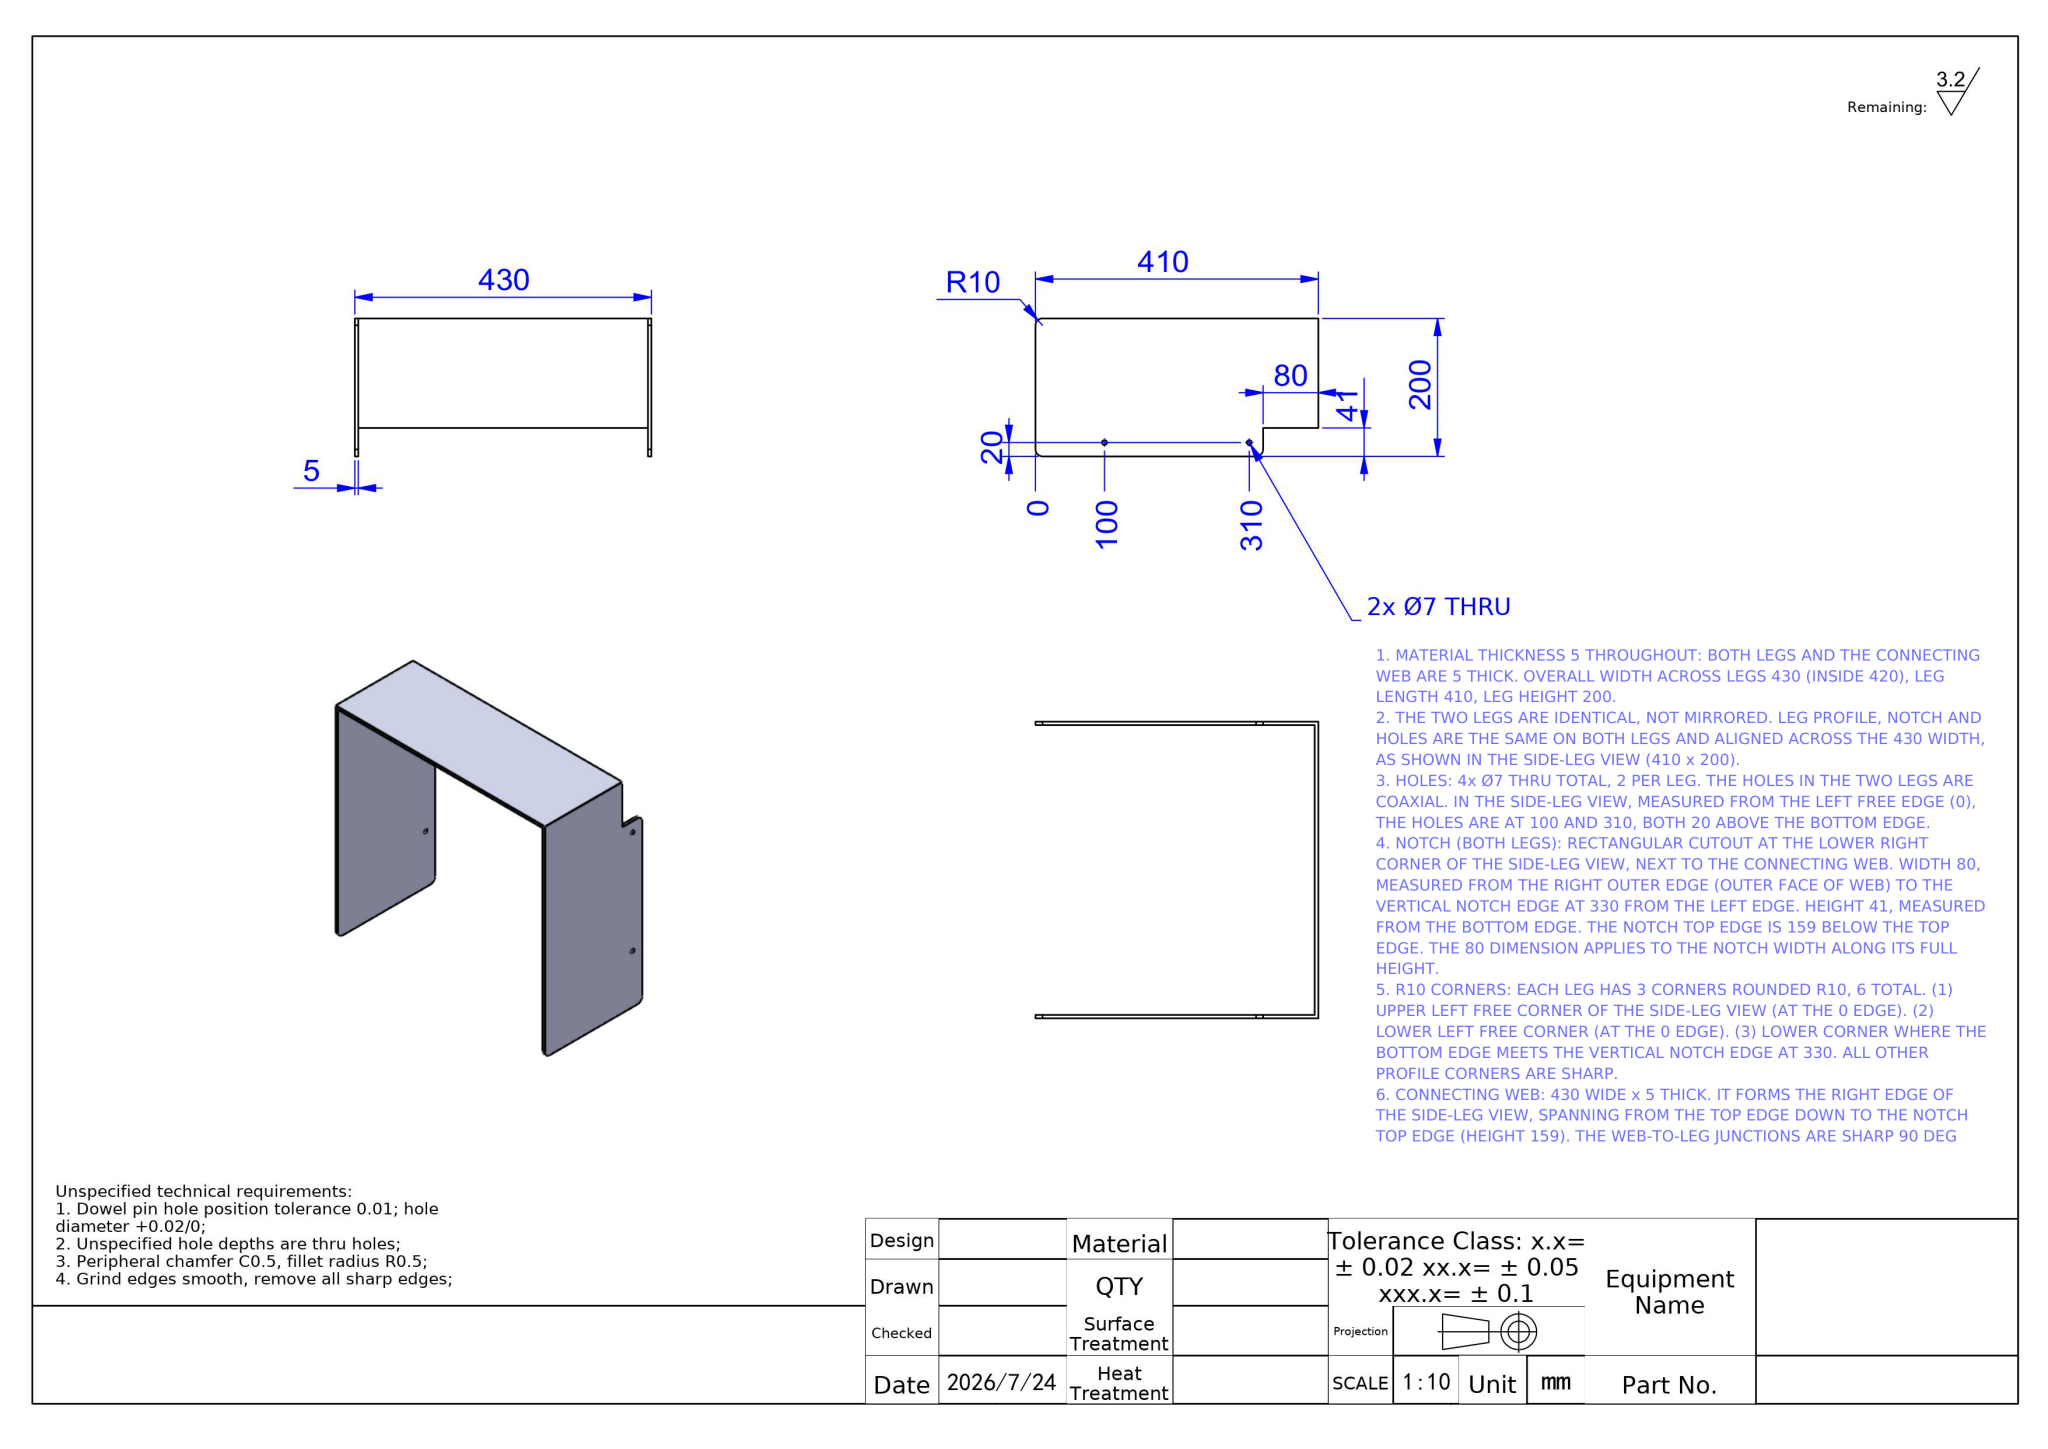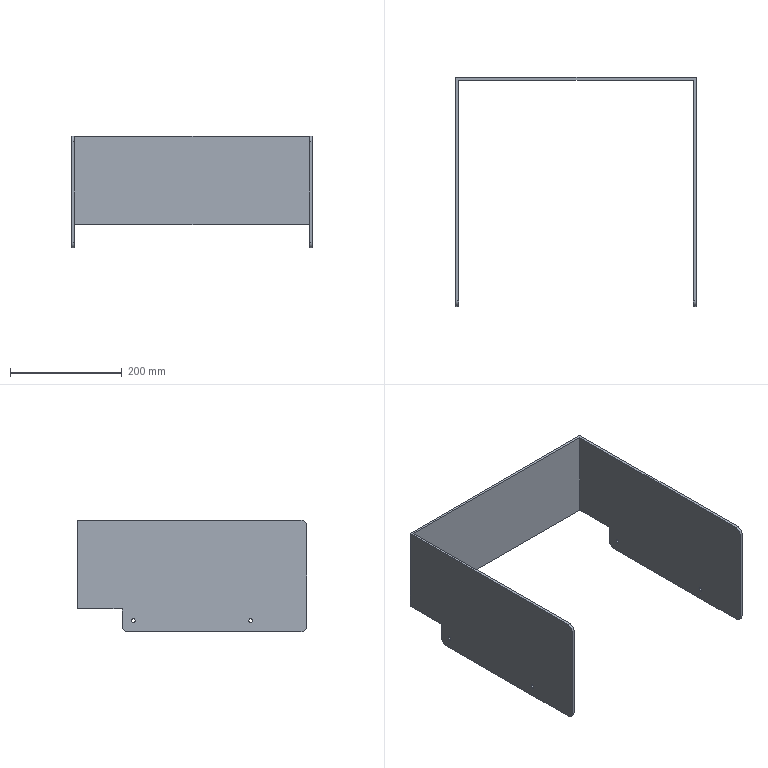Part | NX | mm | Stepped Dual-Tab U-Channel Bracket | 1 solid | 28 faces | box 430 x 410 x 200 mm | volume 1119687 mm3 | cylinder 14 | plane 14 | commonest cylinder face diameters 7 x8 20 x6
STEP:
#1=COLOUR_RGB('',0.7922,0.8196,0.9333);
#2=FILL_AREA_STYLE_COLOUR('',#1);
#3=FILL_AREA_STYLE('',(#2));
#4=SURFACE_STYLE_FILL_AREA(#3);
#5=SURFACE_SIDE_STYLE('',(#4));
#6=SURFACE_STYLE_USAGE(.BOTH.,#5);
#7=PRESENTATION_STYLE_ASSIGNMENT((#6));
#8=CARTESIAN_POINT('',(-210.,105.,-76.5));
#9=VERTEX_POINT('',#8);
#10=CARTESIAN_POINT('',(-210.,105.,-83.5));
#11=VERTEX_POINT('',#10);
#12=CARTESIAN_POINT('',(-210.,105.,-80.));
#13=DIRECTION('',(1.,0.,0.));
#14=DIRECTION('',(0.,1.,0.));
#15=AXIS2_PLACEMENT_3D('',#12,#13,#14);
#16=CIRCLE('',#15,3.5);
#17=EDGE_CURVE('',#9,#11,#16,.T.);
#18=ORIENTED_EDGE('',*,*,#17,.T.);
#19=CARTESIAN_POINT('',(-215.,105.,-83.5));
#20=VERTEX_POINT('',#19);
#21=CARTESIAN_POINT('',(-215.,105.,-83.5));
#22=DIRECTION('',(-1.,0.,0.));
#23=VECTOR('',#22,1000.);
#24=LINE('',#21,#23);
#25=EDGE_CURVE('',#11,#20,#24,.T.);
#26=ORIENTED_EDGE('',*,*,#25,.T.);
#27=CARTESIAN_POINT('',(-215.,105.,-76.5));
#28=VERTEX_POINT('',#27);
#29=CARTESIAN_POINT('',(-215.,105.,-80.));
#30=DIRECTION('',(-1.,0.,0.));
#31=DIRECTION('',(0.,0.,1.));
#32=AXIS2_PLACEMENT_3D('',#29,#30,#31);
#33=CIRCLE('',#32,3.5);
#34=EDGE_CURVE('',#20,#28,#33,.T.);
#35=ORIENTED_EDGE('',*,*,#34,.T.);
#36=CARTESIAN_POINT('',(-215.,105.,-76.5));
#37=DIRECTION('',(-1.,0.,0.));
#38=VECTOR('',#37,1000.);
#39=LINE('',#36,#38);
#40=EDGE_CURVE('',#9,#28,#39,.T.);
#41=ORIENTED_EDGE('',*,*,#40,.F.);
#42=EDGE_LOOP('',(#18,#26,#35,#41));
#43=FACE_OUTER_BOUND('',#42,.T.);
#44=CARTESIAN_POINT('',(-215.,105.,-80.));
#45=DIRECTION('',(-1.,0.,0.));
#46=DIRECTION('',(0.,0.,1.));
#47=AXIS2_PLACEMENT_3D('',#44,#45,#46);
#48=CYLINDRICAL_SURFACE('',#47,3.5);
#49=ADVANCED_FACE('',(#43),#48,.F.);
#50=CARTESIAN_POINT('',(215.,105.,-83.5));
#51=VERTEX_POINT('',#50);
#52=CARTESIAN_POINT('',(215.,105.,-76.5));
#53=VERTEX_POINT('',#52);
#54=CARTESIAN_POINT('',(215.,105.,-80.));
#55=DIRECTION('',(-1.,0.,0.));
#56=DIRECTION('',(0.,0.,1.));
#57=AXIS2_PLACEMENT_3D('',#54,#55,#56);
#58=CIRCLE('',#57,3.5);
#59=EDGE_CURVE('',#51,#53,#58,.T.);
#60=ORIENTED_EDGE('',*,*,#59,.F.);
#61=CARTESIAN_POINT('',(210.,105.,-83.5));
#62=VERTEX_POINT('',#61);
#63=CARTESIAN_POINT('',(-215.,105.,-83.5));
#64=DIRECTION('',(-1.,0.,0.));
#65=VECTOR('',#64,1000.);
#66=LINE('',#63,#65);
#67=EDGE_CURVE('',#51,#62,#66,.T.);
#68=ORIENTED_EDGE('',*,*,#67,.T.);
#69=CARTESIAN_POINT('',(210.,105.,-76.5));
#70=VERTEX_POINT('',#69);
#71=CARTESIAN_POINT('',(210.,105.,-80.));
#72=DIRECTION('',(-1.,-0.,0.));
#73=DIRECTION('',(0.,-1.,0.));
#74=AXIS2_PLACEMENT_3D('',#71,#72,#73);
#75=CIRCLE('',#74,3.5);
#76=EDGE_CURVE('',#62,#70,#75,.T.);
#77=ORIENTED_EDGE('',*,*,#76,.T.);
#78=CARTESIAN_POINT('',(-215.,105.,-76.5));
#79=DIRECTION('',(-1.,0.,0.));
#80=VECTOR('',#79,1000.);
#81=LINE('',#78,#80);
#82=EDGE_CURVE('',#53,#70,#81,.T.);
#83=ORIENTED_EDGE('',*,*,#82,.F.);
#84=EDGE_LOOP('',(#60,#68,#77,#83));
#85=FACE_OUTER_BOUND('',#84,.T.);
#86=CARTESIAN_POINT('',(-215.,105.,-80.));
#87=DIRECTION('',(-1.,0.,0.));
#88=DIRECTION('',(0.,0.,1.));
#89=AXIS2_PLACEMENT_3D('',#86,#87,#88);
#90=CYLINDRICAL_SURFACE('',#89,3.5);
#91=ADVANCED_FACE('',(#85),#90,.F.);
#92=CARTESIAN_POINT('',(215.,-105.,-83.5));
#93=VERTEX_POINT('',#92);
#94=CARTESIAN_POINT('',(215.,-105.,-76.5));
#95=VERTEX_POINT('',#94);
#96=CARTESIAN_POINT('',(215.,-105.,-80.));
#97=DIRECTION('',(-1.,0.,0.));
#98=DIRECTION('',(0.,0.,1.));
#99=AXIS2_PLACEMENT_3D('',#96,#97,#98);
#100=CIRCLE('',#99,3.5);
#101=EDGE_CURVE('',#93,#95,#100,.T.);
#102=ORIENTED_EDGE('',*,*,#101,.F.);
#103=CARTESIAN_POINT('',(210.,-105.,-83.5));
#104=VERTEX_POINT('',#103);
#105=CARTESIAN_POINT('',(-215.,-105.,-83.5));
#106=DIRECTION('',(-1.,0.,0.));
#107=VECTOR('',#106,1000.);
#108=LINE('',#105,#107);
#109=EDGE_CURVE('',#93,#104,#108,.T.);
#110=ORIENTED_EDGE('',*,*,#109,.T.);
#111=CARTESIAN_POINT('',(210.,-105.,-76.5));
#112=VERTEX_POINT('',#111);
#113=CARTESIAN_POINT('',(210.,-105.,-80.));
#114=DIRECTION('',(-1.,-0.,0.));
#115=DIRECTION('',(0.,-1.,0.));
#116=AXIS2_PLACEMENT_3D('',#113,#114,#115);
#117=CIRCLE('',#116,3.5);
#118=EDGE_CURVE('',#104,#112,#117,.T.);
#119=ORIENTED_EDGE('',*,*,#118,.T.);
#120=CARTESIAN_POINT('',(-215.,-105.,-76.5));
#121=DIRECTION('',(-1.,0.,0.));
#122=VECTOR('',#121,1000.);
#123=LINE('',#120,#122);
#124=EDGE_CURVE('',#95,#112,#123,.T.);
#125=ORIENTED_EDGE('',*,*,#124,.F.);
#126=EDGE_LOOP('',(#102,#110,#119,#125));
#127=FACE_OUTER_BOUND('',#126,.T.);
#128=CARTESIAN_POINT('',(-215.,-105.,-80.));
#129=DIRECTION('',(-1.,0.,0.));
#130=DIRECTION('',(0.,0.,1.));
#131=AXIS2_PLACEMENT_3D('',#128,#129,#130);
#132=CYLINDRICAL_SURFACE('',#131,3.5);
#133=ADVANCED_FACE('',(#127),#132,.F.);
#134=CARTESIAN_POINT('',(-210.,-105.,-76.5));
#135=VERTEX_POINT('',#134);
#136=CARTESIAN_POINT('',(-210.,-105.,-83.5));
#137=VERTEX_POINT('',#136);
#138=CARTESIAN_POINT('',(-210.,-105.,-80.));
#139=DIRECTION('',(1.,0.,0.));
#140=DIRECTION('',(0.,1.,0.));
#141=AXIS2_PLACEMENT_3D('',#138,#139,#140);
#142=CIRCLE('',#141,3.5);
#143=EDGE_CURVE('',#135,#137,#142,.T.);
#144=ORIENTED_EDGE('',*,*,#143,.T.);
#145=CARTESIAN_POINT('',(-215.,-105.,-83.5));
#146=VERTEX_POINT('',#145);
#147=CARTESIAN_POINT('',(-215.,-105.,-83.5));
#148=DIRECTION('',(-1.,0.,0.));
#149=VECTOR('',#148,1000.);
#150=LINE('',#147,#149);
#151=EDGE_CURVE('',#137,#146,#150,.T.);
#152=ORIENTED_EDGE('',*,*,#151,.T.);
#153=CARTESIAN_POINT('',(-215.,-105.,-76.5));
#154=VERTEX_POINT('',#153);
#155=CARTESIAN_POINT('',(-215.,-105.,-80.));
#156=DIRECTION('',(-1.,0.,0.));
#157=DIRECTION('',(0.,0.,1.));
#158=AXIS2_PLACEMENT_3D('',#155,#156,#157);
#159=CIRCLE('',#158,3.5);
#160=EDGE_CURVE('',#146,#154,#159,.T.);
#161=ORIENTED_EDGE('',*,*,#160,.T.);
#162=CARTESIAN_POINT('',(-215.,-105.,-76.5));
#163=DIRECTION('',(-1.,0.,0.));
#164=VECTOR('',#163,1000.);
#165=LINE('',#162,#164);
#166=EDGE_CURVE('',#135,#154,#165,.T.);
#167=ORIENTED_EDGE('',*,*,#166,.F.);
#168=EDGE_LOOP('',(#144,#152,#161,#167));
#169=FACE_OUTER_BOUND('',#168,.T.);
#170=CARTESIAN_POINT('',(-215.,-105.,-80.));
#171=DIRECTION('',(-1.,0.,0.));
#172=DIRECTION('',(0.,0.,1.));
#173=AXIS2_PLACEMENT_3D('',#170,#171,#172);
#174=CYLINDRICAL_SURFACE('',#173,3.5);
#175=ADVANCED_FACE('',(#169),#174,.F.);
#176=CARTESIAN_POINT('',(210.,-195.,-100.));
#177=VERTEX_POINT('',#176);
#178=CARTESIAN_POINT('',(210.,115.,-100.));
#179=VERTEX_POINT('',#178);
#180=CARTESIAN_POINT('',(210.,200.,-100.));
#181=DIRECTION('',(-0.,1.,0.));
#182=VECTOR('',#181,1000.);
#183=LINE('',#180,#182);
#184=EDGE_CURVE('',#177,#179,#183,.T.);
#185=ORIENTED_EDGE('',*,*,#184,.T.);
#186=CARTESIAN_POINT('',(215.,115.,-100.));
#187=VERTEX_POINT('',#186);
#188=CARTESIAN_POINT('',(215.,115.,-100.));
#189=DIRECTION('',(1.,-0.,0.));
#190=VECTOR('',#189,1000.);
#191=LINE('',#188,#190);
#192=EDGE_CURVE('',#179,#187,#191,.T.);
#193=ORIENTED_EDGE('',*,*,#192,.T.);
#194=CARTESIAN_POINT('',(215.,-195.,-100.));
#195=VERTEX_POINT('',#194);
#196=CARTESIAN_POINT('',(215.,205.,-100.));
#197=DIRECTION('',(-0.,1.,0.));
#198=VECTOR('',#197,1000.);
#199=LINE('',#196,#198);
#200=EDGE_CURVE('',#195,#187,#199,.T.);
#201=ORIENTED_EDGE('',*,*,#200,.F.);
#202=CARTESIAN_POINT('',(0.,-195.,-100.));
#203=DIRECTION('',(-1.,0.,0.));
#204=VECTOR('',#203,1000.);
#205=LINE('',#202,#204);
#206=EDGE_CURVE('',#195,#177,#205,.T.);
#207=ORIENTED_EDGE('',*,*,#206,.T.);
#208=EDGE_LOOP('',(#185,#193,#201,#207));
#209=FACE_OUTER_BOUND('',#208,.T.);
#210=CARTESIAN_POINT('',(0.,0.,-100.));
#211=DIRECTION('',(0.,0.,1.));
#212=DIRECTION('',(1.,0.,0.));
#213=AXIS2_PLACEMENT_3D('',#210,#211,#212);
#214=PLANE('',#213);
#215=ADVANCED_FACE('',(#209),#214,.F.);
#216=CARTESIAN_POINT('',(215.,-105.,-80.));
#217=DIRECTION('',(-1.,0.,0.));
#218=DIRECTION('',(0.,0.,1.));
#219=AXIS2_PLACEMENT_3D('',#216,#217,#218);
#220=CIRCLE('',#219,3.5);
#221=EDGE_CURVE('',#95,#93,#220,.T.);
#222=ORIENTED_EDGE('',*,*,#221,.T.);
#223=ORIENTED_EDGE('',*,*,#101,.T.);
#224=EDGE_LOOP('',(#222,#223));
#225=FACE_BOUND('',#224,.T.);
#226=CARTESIAN_POINT('',(215.,105.,-80.));
#227=DIRECTION('',(-1.,0.,0.));
#228=DIRECTION('',(0.,0.,1.));
#229=AXIS2_PLACEMENT_3D('',#226,#227,#228);
#230=CIRCLE('',#229,3.5);
#231=EDGE_CURVE('',#53,#51,#230,.T.);
#232=ORIENTED_EDGE('',*,*,#231,.T.);
#233=ORIENTED_EDGE('',*,*,#59,.T.);
#234=EDGE_LOOP('',(#232,#233));
#235=FACE_BOUND('',#234,.T.);
#236=CARTESIAN_POINT('',(215.,-195.,100.));
#237=VERTEX_POINT('',#236);
#238=CARTESIAN_POINT('',(215.,205.,100.));
#239=VERTEX_POINT('',#238);
#240=CARTESIAN_POINT('',(215.,205.,100.));
#241=DIRECTION('',(-0.,1.,0.));
#242=VECTOR('',#241,1000.);
#243=LINE('',#240,#242);
#244=EDGE_CURVE('',#237,#239,#243,.T.);
#245=ORIENTED_EDGE('',*,*,#244,.F.);
#246=CARTESIAN_POINT('',(215.,-205.,90.));
#247=VERTEX_POINT('',#246);
#248=CARTESIAN_POINT('',(215.,-195.,90.));
#249=DIRECTION('',(1.,0.,0.));
#250=DIRECTION('',(0.,-1.,0.));
#251=AXIS2_PLACEMENT_3D('',#248,#249,#250);
#252=CIRCLE('',#251,10.);
#253=EDGE_CURVE('',#237,#247,#252,.T.);
#254=ORIENTED_EDGE('',*,*,#253,.T.);
#255=CARTESIAN_POINT('',(215.,-205.,-90.));
#256=VERTEX_POINT('',#255);
#257=CARTESIAN_POINT('',(215.,-205.,100.));
#258=DIRECTION('',(0.,0.,-1.));
#259=VECTOR('',#258,1000.);
#260=LINE('',#257,#259);
#261=EDGE_CURVE('',#247,#256,#260,.T.);
#262=ORIENTED_EDGE('',*,*,#261,.T.);
#263=CARTESIAN_POINT('',(215.,-195.,-90.));
#264=DIRECTION('',(1.,0.,0.));
#265=DIRECTION('',(0.,-1.,0.));
#266=AXIS2_PLACEMENT_3D('',#263,#264,#265);
#267=CIRCLE('',#266,10.);
#268=EDGE_CURVE('',#256,#195,#267,.T.);
#269=ORIENTED_EDGE('',*,*,#268,.T.);
#270=ORIENTED_EDGE('',*,*,#200,.T.);
#271=CARTESIAN_POINT('',(215.,125.,-90.));
#272=VERTEX_POINT('',#271);
#273=CARTESIAN_POINT('',(215.,115.,-90.));
#274=DIRECTION('',(1.,0.,0.));
#275=DIRECTION('',(0.,-1.,0.));
#276=AXIS2_PLACEMENT_3D('',#273,#274,#275);
#277=CIRCLE('',#276,10.);
#278=EDGE_CURVE('',#187,#272,#277,.T.);
#279=ORIENTED_EDGE('',*,*,#278,.T.);
#280=CARTESIAN_POINT('',(215.,125.,-59.));
#281=VERTEX_POINT('',#280);
#282=CARTESIAN_POINT('',(215.,125.,-100.));
#283=DIRECTION('',(0.,0.,1.));
#284=VECTOR('',#283,1000.);
#285=LINE('',#282,#284);
#286=EDGE_CURVE('',#272,#281,#285,.T.);
#287=ORIENTED_EDGE('',*,*,#286,.T.);
#288=CARTESIAN_POINT('',(215.,205.,-59.));
#289=VERTEX_POINT('',#288);
#290=CARTESIAN_POINT('',(215.,205.,-59.));
#291=DIRECTION('',(0.,1.,0.));
#292=VECTOR('',#291,1000.);
#293=LINE('',#290,#292);
#294=EDGE_CURVE('',#281,#289,#293,.T.);
#295=ORIENTED_EDGE('',*,*,#294,.T.);
#296=CARTESIAN_POINT('',(215.,205.,100.));
#297=DIRECTION('',(0.,0.,-1.));
#298=VECTOR('',#297,1000.);
#299=LINE('',#296,#298);
#300=EDGE_CURVE('',#239,#289,#299,.T.);
#301=ORIENTED_EDGE('',*,*,#300,.F.);
#302=EDGE_LOOP('',(#245,#254,#262,#269,#270,#279,#287,#295,#301));
#303=FACE_OUTER_BOUND('',#302,.T.);
#304=CARTESIAN_POINT('',(215.,205.,100.));
#305=DIRECTION('',(-1.,-0.,0.));
#306=DIRECTION('',(0.,-1.,0.));
#307=AXIS2_PLACEMENT_3D('',#304,#305,#306);
#308=PLANE('',#307);
#309=ADVANCED_FACE('',(#225,#235,#303),#308,.F.);
#310=ORIENTED_EDGE('',*,*,#300,.T.);
#311=CARTESIAN_POINT('',(-215.,205.,-59.));
#312=VERTEX_POINT('',#311);
#313=CARTESIAN_POINT('',(-120.106,205.,-59.));
#314=DIRECTION('',(-1.,-0.,0.));
#315=VECTOR('',#314,1000.);
#316=LINE('',#313,#315);
#317=EDGE_CURVE('',#289,#312,#316,.T.);
#318=ORIENTED_EDGE('',*,*,#317,.T.);
#319=CARTESIAN_POINT('',(-215.,205.,100.));
#320=VERTEX_POINT('',#319);
#321=CARTESIAN_POINT('',(-215.,205.,100.));
#322=DIRECTION('',(0.,0.,-1.));
#323=VECTOR('',#322,1000.);
#324=LINE('',#321,#323);
#325=EDGE_CURVE('',#320,#312,#324,.T.);
#326=ORIENTED_EDGE('',*,*,#325,.F.);
#327=CARTESIAN_POINT('',(-215.,205.,100.));
#328=DIRECTION('',(-1.,0.,0.));
#329=VECTOR('',#328,1000.);
#330=LINE('',#327,#329);
#331=EDGE_CURVE('',#239,#320,#330,.T.);
#332=ORIENTED_EDGE('',*,*,#331,.F.);
#333=EDGE_LOOP('',(#310,#318,#326,#332));
#334=FACE_OUTER_BOUND('',#333,.T.);
#335=CARTESIAN_POINT('',(-215.,205.,100.));
#336=DIRECTION('',(0.,-1.,0.));
#337=DIRECTION('',(0.,0.,-1.));
#338=AXIS2_PLACEMENT_3D('',#335,#336,#337);
#339=PLANE('',#338);
#340=ADVANCED_FACE('',(#334),#339,.F.);
#341=CARTESIAN_POINT('',(210.,105.,-80.));
#342=DIRECTION('',(-1.,-0.,0.));
#343=DIRECTION('',(0.,-1.,0.));
#344=AXIS2_PLACEMENT_3D('',#341,#342,#343);
#345=CIRCLE('',#344,3.5);
#346=EDGE_CURVE('',#70,#62,#345,.T.);
#347=ORIENTED_EDGE('',*,*,#346,.F.);
#348=ORIENTED_EDGE('',*,*,#76,.F.);
#349=EDGE_LOOP('',(#347,#348));
#350=FACE_BOUND('',#349,.T.);
#351=CARTESIAN_POINT('',(210.,-105.,-80.));
#352=DIRECTION('',(-1.,-0.,0.));
#353=DIRECTION('',(0.,-1.,0.));
#354=AXIS2_PLACEMENT_3D('',#351,#352,#353);
#355=CIRCLE('',#354,3.5);
#356=EDGE_CURVE('',#112,#104,#355,.T.);
#357=ORIENTED_EDGE('',*,*,#356,.F.);
#358=ORIENTED_EDGE('',*,*,#118,.F.);
#359=EDGE_LOOP('',(#357,#358));
#360=FACE_BOUND('',#359,.T.);
#361=CARTESIAN_POINT('',(210.,-205.,90.));
#362=VERTEX_POINT('',#361);
#363=CARTESIAN_POINT('',(210.,-205.,-90.));
#364=VERTEX_POINT('',#363);
#365=CARTESIAN_POINT('',(210.,-205.,100.));
#366=DIRECTION('',(0.,0.,-1.));
#367=VECTOR('',#366,1000.);
#368=LINE('',#365,#367);
#369=EDGE_CURVE('',#362,#364,#368,.T.);
#370=ORIENTED_EDGE('',*,*,#369,.F.);
#371=CARTESIAN_POINT('',(210.,-195.,100.));
#372=VERTEX_POINT('',#371);
#373=CARTESIAN_POINT('',(210.,-195.,90.));
#374=DIRECTION('',(-1.,-0.,0.));
#375=DIRECTION('',(0.,-1.,0.));
#376=AXIS2_PLACEMENT_3D('',#373,#374,#375);
#377=CIRCLE('',#376,10.);
#378=EDGE_CURVE('',#362,#372,#377,.T.);
#379=ORIENTED_EDGE('',*,*,#378,.T.);
#380=CARTESIAN_POINT('',(210.,200.,100.));
#381=VERTEX_POINT('',#380);
#382=CARTESIAN_POINT('',(210.,200.,100.));
#383=DIRECTION('',(-0.,1.,0.));
#384=VECTOR('',#383,1000.);
#385=LINE('',#382,#384);
#386=EDGE_CURVE('',#372,#381,#385,.T.);
#387=ORIENTED_EDGE('',*,*,#386,.T.);
#388=CARTESIAN_POINT('',(210.,200.,-59.));
#389=VERTEX_POINT('',#388);
#390=CARTESIAN_POINT('',(210.,200.,100.));
#391=DIRECTION('',(0.,0.,-1.));
#392=VECTOR('',#391,1000.);
#393=LINE('',#390,#392);
#394=EDGE_CURVE('',#381,#389,#393,.T.);
#395=ORIENTED_EDGE('',*,*,#394,.T.);
#396=CARTESIAN_POINT('',(210.,125.,-59.));
#397=VERTEX_POINT('',#396);
#398=CARTESIAN_POINT('',(210.,200.,-59.));
#399=DIRECTION('',(0.,-1.,0.));
#400=VECTOR('',#399,1000.);
#401=LINE('',#398,#400);
#402=EDGE_CURVE('',#389,#397,#401,.T.);
#403=ORIENTED_EDGE('',*,*,#402,.T.);
#404=CARTESIAN_POINT('',(210.,125.,-90.));
#405=VERTEX_POINT('',#404);
#406=CARTESIAN_POINT('',(210.,125.,100.));
#407=DIRECTION('',(0.,0.,-1.));
#408=VECTOR('',#407,1000.);
#409=LINE('',#406,#408);
#410=EDGE_CURVE('',#397,#405,#409,.T.);
#411=ORIENTED_EDGE('',*,*,#410,.T.);
#412=CARTESIAN_POINT('',(210.,115.,-90.));
#413=DIRECTION('',(-1.,-0.,0.));
#414=DIRECTION('',(0.,-1.,0.));
#415=AXIS2_PLACEMENT_3D('',#412,#413,#414);
#416=CIRCLE('',#415,10.);
#417=EDGE_CURVE('',#405,#179,#416,.T.);
#418=ORIENTED_EDGE('',*,*,#417,.T.);
#419=ORIENTED_EDGE('',*,*,#184,.F.);
#420=CARTESIAN_POINT('',(210.,-195.,-90.));
#421=DIRECTION('',(-1.,-0.,0.));
#422=DIRECTION('',(0.,-1.,0.));
#423=AXIS2_PLACEMENT_3D('',#420,#421,#422);
#424=CIRCLE('',#423,10.);
#425=EDGE_CURVE('',#177,#364,#424,.T.);
#426=ORIENTED_EDGE('',*,*,#425,.T.);
#427=EDGE_LOOP('',(#370,#379,#387,#395,#403,#411,#418,#419,#426));
#428=FACE_OUTER_BOUND('',#427,.T.);
#429=CARTESIAN_POINT('',(210.,200.,100.));
#430=DIRECTION('',(-1.,-0.,0.));
#431=DIRECTION('',(0.,-1.,0.));
#432=AXIS2_PLACEMENT_3D('',#429,#430,#431);
#433=PLANE('',#432);
#434=ADVANCED_FACE('',(#350,#360,#428),#433,.T.);
#435=CARTESIAN_POINT('',(-210.,200.,100.));
#436=VERTEX_POINT('',#435);
#437=CARTESIAN_POINT('',(-210.,200.,-59.));
#438=VERTEX_POINT('',#437);
#439=CARTESIAN_POINT('',(-210.,200.,100.));
#440=DIRECTION('',(0.,0.,-1.));
#441=VECTOR('',#440,1000.);
#442=LINE('',#439,#441);
#443=EDGE_CURVE('',#436,#438,#442,.T.);
#444=ORIENTED_EDGE('',*,*,#443,.T.);
#445=CARTESIAN_POINT('',(-210.,200.,-59.));
#446=DIRECTION('',(1.,0.,0.));
#447=VECTOR('',#446,1000.);
#448=LINE('',#445,#447);
#449=EDGE_CURVE('',#438,#389,#448,.T.);
#450=ORIENTED_EDGE('',*,*,#449,.T.);
#451=ORIENTED_EDGE('',*,*,#394,.F.);
#452=CARTESIAN_POINT('',(-210.,200.,100.));
#453=DIRECTION('',(-1.,0.,0.));
#454=VECTOR('',#453,1000.);
#455=LINE('',#452,#454);
#456=EDGE_CURVE('',#381,#436,#455,.T.);
#457=ORIENTED_EDGE('',*,*,#456,.T.);
#458=EDGE_LOOP('',(#444,#450,#451,#457));
#459=FACE_OUTER_BOUND('',#458,.T.);
#460=CARTESIAN_POINT('',(-210.,200.,100.));
#461=DIRECTION('',(0.,-1.,0.));
#462=DIRECTION('',(0.,0.,-1.));
#463=AXIS2_PLACEMENT_3D('',#460,#461,#462);
#464=PLANE('',#463);
#465=ADVANCED_FACE('',(#459),#464,.T.);
#466=ORIENTED_EDGE('',*,*,#261,.F.);
#467=CARTESIAN_POINT('',(210.,-205.,90.));
#468=DIRECTION('',(-1.,0.,0.));
#469=VECTOR('',#468,1000.);
#470=LINE('',#467,#469);
#471=EDGE_CURVE('',#247,#362,#470,.T.);
#472=ORIENTED_EDGE('',*,*,#471,.T.);
#473=ORIENTED_EDGE('',*,*,#369,.T.);
#474=CARTESIAN_POINT('',(-215.,-205.,-90.));
#475=DIRECTION('',(1.,0.,0.));
#476=VECTOR('',#475,1000.);
#477=LINE('',#474,#476);
#478=EDGE_CURVE('',#364,#256,#477,.T.);
#479=ORIENTED_EDGE('',*,*,#478,.T.);
#480=EDGE_LOOP('',(#466,#472,#473,#479));
#481=FACE_OUTER_BOUND('',#480,.T.);
#482=CARTESIAN_POINT('',(-215.,-205.,100.));
#483=DIRECTION('',(0.,1.,0.));
#484=DIRECTION('',(0.,0.,1.));
#485=AXIS2_PLACEMENT_3D('',#482,#483,#484);
#486=PLANE('',#485);
#487=ADVANCED_FACE('',(#481),#486,.F.);
#488=ORIENTED_EDGE('',*,*,#386,.F.);
#489=CARTESIAN_POINT('',(215.,-195.,100.));
#490=DIRECTION('',(1.,0.,0.));
#491=VECTOR('',#490,1000.);
#492=LINE('',#489,#491);
#493=EDGE_CURVE('',#372,#237,#492,.T.);
#494=ORIENTED_EDGE('',*,*,#493,.T.);
#495=ORIENTED_EDGE('',*,*,#244,.T.);
#496=ORIENTED_EDGE('',*,*,#331,.T.);
#497=CARTESIAN_POINT('',(-215.,-195.,100.));
#498=VERTEX_POINT('',#497);
#499=CARTESIAN_POINT('',(-215.,205.,100.));
#500=DIRECTION('',(0.,-1.,0.));
#501=VECTOR('',#500,1000.);
#502=LINE('',#499,#501);
#503=EDGE_CURVE('',#320,#498,#502,.T.);
#504=ORIENTED_EDGE('',*,*,#503,.T.);
#505=CARTESIAN_POINT('',(-210.,-195.,100.));
#506=VERTEX_POINT('',#505);
#507=CARTESIAN_POINT('',(-210.,-195.,100.));
#508=DIRECTION('',(1.,0.,0.));
#509=VECTOR('',#508,1000.);
#510=LINE('',#507,#509);
#511=EDGE_CURVE('',#498,#506,#510,.T.);
#512=ORIENTED_EDGE('',*,*,#511,.T.);
#513=CARTESIAN_POINT('',(-210.,200.,100.));
#514=DIRECTION('',(0.,-1.,0.));
#515=VECTOR('',#514,1000.);
#516=LINE('',#513,#515);
#517=EDGE_CURVE('',#436,#506,#516,.T.);
#518=ORIENTED_EDGE('',*,*,#517,.F.);
#519=ORIENTED_EDGE('',*,*,#456,.F.);
#520=EDGE_LOOP('',(#488,#494,#495,#496,#504,#512,#518,#519));
#521=FACE_OUTER_BOUND('',#520,.T.);
#522=CARTESIAN_POINT('',(0.,0.,100.));
#523=DIRECTION('',(0.,0.,1.));
#524=DIRECTION('',(1.,0.,0.));
#525=AXIS2_PLACEMENT_3D('',#522,#523,#524);
#526=PLANE('',#525);
#527=ADVANCED_FACE('',(#521),#526,.T.);
#528=CARTESIAN_POINT('',(-215.,115.,-100.));
#529=VERTEX_POINT('',#528);
#530=CARTESIAN_POINT('',(-215.,-195.,-100.));
#531=VERTEX_POINT('',#530);
#532=CARTESIAN_POINT('',(-215.,205.,-100.));
#533=DIRECTION('',(0.,-1.,0.));
#534=VECTOR('',#533,1000.);
#535=LINE('',#532,#534);
#536=EDGE_CURVE('',#529,#531,#535,.T.);
#537=ORIENTED_EDGE('',*,*,#536,.F.);
#538=CARTESIAN_POINT('',(-210.,115.,-100.));
#539=VERTEX_POINT('',#538);
#540=CARTESIAN_POINT('',(-0.,115.,-100.));
#541=DIRECTION('',(1.,0.,0.));
#542=VECTOR('',#541,1000.);
#543=LINE('',#540,#542);
#544=EDGE_CURVE('',#529,#539,#543,.T.);
#545=ORIENTED_EDGE('',*,*,#544,.T.);
#546=CARTESIAN_POINT('',(-210.,-195.,-100.));
#547=VERTEX_POINT('',#546);
#548=CARTESIAN_POINT('',(-210.,200.,-100.));
#549=DIRECTION('',(0.,-1.,0.));
#550=VECTOR('',#549,1000.);
#551=LINE('',#548,#550);
#552=EDGE_CURVE('',#539,#547,#551,.T.);
#553=ORIENTED_EDGE('',*,*,#552,.T.);
#554=CARTESIAN_POINT('',(0.,-195.,-100.));
#555=DIRECTION('',(-1.,0.,0.));
#556=VECTOR('',#555,1000.);
#557=LINE('',#554,#556);
#558=EDGE_CURVE('',#547,#531,#557,.T.);
#559=ORIENTED_EDGE('',*,*,#558,.T.);
#560=EDGE_LOOP('',(#537,#545,#553,#559));
#561=FACE_OUTER_BOUND('',#560,.T.);
#562=CARTESIAN_POINT('',(0.,0.,-100.));
#563=DIRECTION('',(0.,0.,1.));
#564=DIRECTION('',(1.,0.,0.));
#565=AXIS2_PLACEMENT_3D('',#562,#563,#564);
#566=PLANE('',#565);
#567=ADVANCED_FACE('',(#561),#566,.F.);
#568=CARTESIAN_POINT('',(-215.,105.,-80.));
#569=DIRECTION('',(-1.,0.,0.));
#570=DIRECTION('',(0.,0.,1.));
#571=AXIS2_PLACEMENT_3D('',#568,#569,#570);
#572=CIRCLE('',#571,3.5);
#573=EDGE_CURVE('',#28,#20,#572,.T.);
#574=ORIENTED_EDGE('',*,*,#573,.F.);
#575=ORIENTED_EDGE('',*,*,#34,.F.);
#576=EDGE_LOOP('',(#574,#575));
#577=FACE_BOUND('',#576,.T.);
#578=CARTESIAN_POINT('',(-215.,-105.,-80.));
#579=DIRECTION('',(-1.,0.,0.));
#580=DIRECTION('',(0.,0.,1.));
#581=AXIS2_PLACEMENT_3D('',#578,#579,#580);
#582=CIRCLE('',#581,3.5);
#583=EDGE_CURVE('',#154,#146,#582,.T.);
#584=ORIENTED_EDGE('',*,*,#583,.F.);
#585=ORIENTED_EDGE('',*,*,#160,.F.);
#586=EDGE_LOOP('',(#584,#585));
#587=FACE_BOUND('',#586,.T.);
#588=CARTESIAN_POINT('',(-215.,125.,-90.));
#589=VERTEX_POINT('',#588);
#590=CARTESIAN_POINT('',(-215.,125.,-59.));
#591=VERTEX_POINT('',#590);
#592=CARTESIAN_POINT('',(-215.,125.,-100.));
#593=DIRECTION('',(0.,0.,1.));
#594=VECTOR('',#593,1000.);
#595=LINE('',#592,#594);
#596=EDGE_CURVE('',#589,#591,#595,.T.);
#597=ORIENTED_EDGE('',*,*,#596,.F.);
#598=CARTESIAN_POINT('',(-215.,115.,-90.));
#599=DIRECTION('',(-1.,-0.,0.));
#600=DIRECTION('',(0.,1.,0.));
#601=AXIS2_PLACEMENT_3D('',#598,#599,#600);
#602=CIRCLE('',#601,10.);
#603=EDGE_CURVE('',#589,#529,#602,.T.);
#604=ORIENTED_EDGE('',*,*,#603,.T.);
#605=ORIENTED_EDGE('',*,*,#536,.T.);
#606=CARTESIAN_POINT('',(-215.,-205.,-90.));
#607=VERTEX_POINT('',#606);
#608=CARTESIAN_POINT('',(-215.,-195.,-90.));
#609=DIRECTION('',(-1.,-0.,0.));
#610=DIRECTION('',(0.,1.,0.));
#611=AXIS2_PLACEMENT_3D('',#608,#609,#610);
#612=CIRCLE('',#611,10.);
#613=EDGE_CURVE('',#531,#607,#612,.T.);
#614=ORIENTED_EDGE('',*,*,#613,.T.);
#615=CARTESIAN_POINT('',(-215.,-205.,90.));
#616=VERTEX_POINT('',#615);
#617=CARTESIAN_POINT('',(-215.,-205.,100.));
#618=DIRECTION('',(0.,0.,-1.));
#619=VECTOR('',#618,1000.);
#620=LINE('',#617,#619);
#621=EDGE_CURVE('',#616,#607,#620,.T.);
#622=ORIENTED_EDGE('',*,*,#621,.F.);
#623=CARTESIAN_POINT('',(-215.,-195.,90.));
#624=DIRECTION('',(-1.,-0.,0.));
#625=DIRECTION('',(0.,1.,0.));
#626=AXIS2_PLACEMENT_3D('',#623,#624,#625);
#627=CIRCLE('',#626,10.);
#628=EDGE_CURVE('',#616,#498,#627,.T.);
#629=ORIENTED_EDGE('',*,*,#628,.T.);
#630=ORIENTED_EDGE('',*,*,#503,.F.);
#631=ORIENTED_EDGE('',*,*,#325,.T.);
#632=CARTESIAN_POINT('',(-215.,205.,-59.));
#633=DIRECTION('',(0.,1.,0.));
#634=VECTOR('',#633,1000.);
#635=LINE('',#632,#634);
#636=EDGE_CURVE('',#591,#312,#635,.T.);
#637=ORIENTED_EDGE('',*,*,#636,.F.);
#638=EDGE_LOOP('',(#597,#604,#605,#614,#622,#629,#630,#631,#637));
#639=FACE_OUTER_BOUND('',#638,.T.);
#640=CARTESIAN_POINT('',(-215.,205.,100.));
#641=DIRECTION('',(1.,0.,0.));
#642=DIRECTION('',(-0.,1.,0.));
#643=AXIS2_PLACEMENT_3D('',#640,#641,#642);
#644=PLANE('',#643);
#645=ADVANCED_FACE('',(#577,#587,#639),#644,.F.);
#646=ORIENTED_EDGE('',*,*,#621,.T.);
#647=CARTESIAN_POINT('',(-210.,-205.,-90.));
#648=VERTEX_POINT('',#647);
#649=CARTESIAN_POINT('',(-215.,-205.,-90.));
#650=DIRECTION('',(1.,0.,0.));
#651=VECTOR('',#650,1000.);
#652=LINE('',#649,#651);
#653=EDGE_CURVE('',#607,#648,#652,.T.);
#654=ORIENTED_EDGE('',*,*,#653,.T.);
#655=CARTESIAN_POINT('',(-210.,-205.,90.));
#656=VERTEX_POINT('',#655);
#657=CARTESIAN_POINT('',(-210.,-205.,-100.));
#658=DIRECTION('',(0.,0.,1.));
#659=VECTOR('',#658,1000.);
#660=LINE('',#657,#659);
#661=EDGE_CURVE('',#648,#656,#660,.T.);
#662=ORIENTED_EDGE('',*,*,#661,.T.);
#663=CARTESIAN_POINT('',(-215.,-205.,90.));
#664=DIRECTION('',(-1.,0.,0.));
#665=VECTOR('',#664,1000.);
#666=LINE('',#663,#665);
#667=EDGE_CURVE('',#656,#616,#666,.T.);
#668=ORIENTED_EDGE('',*,*,#667,.T.);
#669=EDGE_LOOP('',(#646,#654,#662,#668));
#670=FACE_OUTER_BOUND('',#669,.T.);
#671=CARTESIAN_POINT('',(-215.,-205.,100.));
#672=DIRECTION('',(0.,1.,0.));
#673=DIRECTION('',(0.,0.,1.));
#674=AXIS2_PLACEMENT_3D('',#671,#672,#673);
#675=PLANE('',#674);
#676=ADVANCED_FACE('',(#670),#675,.F.);
#677=ORIENTED_EDGE('',*,*,#552,.F.);
#678=CARTESIAN_POINT('',(-210.,125.,-90.));
#679=VERTEX_POINT('',#678);
#680=CARTESIAN_POINT('',(-210.,115.,-90.));
#681=DIRECTION('',(1.,0.,0.));
#682=DIRECTION('',(0.,1.,0.));
#683=AXIS2_PLACEMENT_3D('',#680,#681,#682);
#684=CIRCLE('',#683,10.);
#685=EDGE_CURVE('',#539,#679,#684,.T.);
#686=ORIENTED_EDGE('',*,*,#685,.T.);
#687=CARTESIAN_POINT('',(-210.,125.,-59.));
#688=VERTEX_POINT('',#687);
#689=CARTESIAN_POINT('',(-210.,125.,-100.));
#690=DIRECTION('',(0.,0.,1.));
#691=VECTOR('',#690,1000.);
#692=LINE('',#689,#691);
#693=EDGE_CURVE('',#679,#688,#692,.T.);
#694=ORIENTED_EDGE('',*,*,#693,.T.);
#695=CARTESIAN_POINT('',(-210.,205.,-59.));
#696=DIRECTION('',(-0.,1.,0.));
#697=VECTOR('',#696,1000.);
#698=LINE('',#695,#697);
#699=EDGE_CURVE('',#688,#438,#698,.T.);
#700=ORIENTED_EDGE('',*,*,#699,.T.);
#701=ORIENTED_EDGE('',*,*,#443,.F.);
#702=ORIENTED_EDGE('',*,*,#517,.T.);
#703=CARTESIAN_POINT('',(-210.,-195.,90.));
#704=DIRECTION('',(1.,0.,0.));
#705=DIRECTION('',(0.,1.,0.));
#706=AXIS2_PLACEMENT_3D('',#703,#704,#705);
#707=CIRCLE('',#706,10.);
#708=EDGE_CURVE('',#506,#656,#707,.T.);
#709=ORIENTED_EDGE('',*,*,#708,.T.);
#710=ORIENTED_EDGE('',*,*,#661,.F.);
#711=CARTESIAN_POINT('',(-210.,-195.,-90.));
#712=DIRECTION('',(1.,0.,0.));
#713=DIRECTION('',(0.,1.,0.));
#714=AXIS2_PLACEMENT_3D('',#711,#712,#713);
#715=CIRCLE('',#714,10.);
#716=EDGE_CURVE('',#648,#547,#715,.T.);
#717=ORIENTED_EDGE('',*,*,#716,.T.);
#718=EDGE_LOOP('',(#677,#686,#694,#700,#701,#702,#709,#710,#717));
#719=FACE_OUTER_BOUND('',#718,.T.);
#720=ORIENTED_EDGE('',*,*,#17,.F.);
#721=CARTESIAN_POINT('',(-210.,105.,-80.));
#722=DIRECTION('',(1.,0.,0.));
#723=DIRECTION('',(0.,1.,0.));
#724=AXIS2_PLACEMENT_3D('',#721,#722,#723);
#725=CIRCLE('',#724,3.5);
#726=EDGE_CURVE('',#11,#9,#725,.T.);
#727=ORIENTED_EDGE('',*,*,#726,.F.);
#728=EDGE_LOOP('',(#720,#727));
#729=FACE_BOUND('',#728,.T.);
#730=ORIENTED_EDGE('',*,*,#143,.F.);
#731=CARTESIAN_POINT('',(-210.,-105.,-80.));
#732=DIRECTION('',(1.,0.,0.));
#733=DIRECTION('',(0.,1.,0.));
#734=AXIS2_PLACEMENT_3D('',#731,#732,#733);
#735=CIRCLE('',#734,3.5);
#736=EDGE_CURVE('',#137,#135,#735,.T.);
#737=ORIENTED_EDGE('',*,*,#736,.F.);
#738=EDGE_LOOP('',(#730,#737));
#739=FACE_BOUND('',#738,.T.);
#740=CARTESIAN_POINT('',(-210.,200.,100.));
#741=DIRECTION('',(1.,0.,0.));
#742=DIRECTION('',(-0.,1.,0.));
#743=AXIS2_PLACEMENT_3D('',#740,#741,#742);
#744=PLANE('',#743);
#745=ADVANCED_FACE('',(#719,#729,#739),#744,.T.);
#746=ORIENTED_EDGE('',*,*,#151,.F.);
#747=ORIENTED_EDGE('',*,*,#736,.T.);
#748=ORIENTED_EDGE('',*,*,#166,.T.);
#749=ORIENTED_EDGE('',*,*,#583,.T.);
#750=EDGE_LOOP('',(#746,#747,#748,#749));
#751=FACE_OUTER_BOUND('',#750,.T.);
#752=CARTESIAN_POINT('',(-215.,-105.,-80.));
#753=DIRECTION('',(-1.,0.,0.));
#754=DIRECTION('',(0.,0.,1.));
#755=AXIS2_PLACEMENT_3D('',#752,#753,#754);
#756=CYLINDRICAL_SURFACE('',#755,3.5);
#757=ADVANCED_FACE('',(#751),#756,.F.);
#758=ORIENTED_EDGE('',*,*,#109,.F.);
#759=ORIENTED_EDGE('',*,*,#221,.F.);
#760=ORIENTED_EDGE('',*,*,#124,.T.);
#761=ORIENTED_EDGE('',*,*,#356,.T.);
#762=EDGE_LOOP('',(#758,#759,#760,#761));
#763=FACE_OUTER_BOUND('',#762,.T.);
#764=CARTESIAN_POINT('',(-215.,-105.,-80.));
#765=DIRECTION('',(-1.,0.,0.));
#766=DIRECTION('',(0.,0.,1.));
#767=AXIS2_PLACEMENT_3D('',#764,#765,#766);
#768=CYLINDRICAL_SURFACE('',#767,3.5);
#769=ADVANCED_FACE('',(#763),#768,.F.);
#770=ORIENTED_EDGE('',*,*,#67,.F.);
#771=ORIENTED_EDGE('',*,*,#231,.F.);
#772=ORIENTED_EDGE('',*,*,#82,.T.);
#773=ORIENTED_EDGE('',*,*,#346,.T.);
#774=EDGE_LOOP('',(#770,#771,#772,#773));
#775=FACE_OUTER_BOUND('',#774,.T.);
#776=CARTESIAN_POINT('',(-215.,105.,-80.));
#777=DIRECTION('',(-1.,0.,0.));
#778=DIRECTION('',(0.,0.,1.));
#779=AXIS2_PLACEMENT_3D('',#776,#777,#778);
#780=CYLINDRICAL_SURFACE('',#779,3.5);
#781=ADVANCED_FACE('',(#775),#780,.F.);
#782=ORIENTED_EDGE('',*,*,#25,.F.);
#783=ORIENTED_EDGE('',*,*,#726,.T.);
#784=ORIENTED_EDGE('',*,*,#40,.T.);
#785=ORIENTED_EDGE('',*,*,#573,.T.);
#786=EDGE_LOOP('',(#782,#783,#784,#785));
#787=FACE_OUTER_BOUND('',#786,.T.);
#788=CARTESIAN_POINT('',(-215.,105.,-80.));
#789=DIRECTION('',(-1.,0.,0.));
#790=DIRECTION('',(0.,0.,1.));
#791=AXIS2_PLACEMENT_3D('',#788,#789,#790);
#792=CYLINDRICAL_SURFACE('',#791,3.5);
#793=ADVANCED_FACE('',(#787),#792,.F.);
#794=ORIENTED_EDGE('',*,*,#693,.F.);
#795=CARTESIAN_POINT('',(-120.106,125.,-90.));
#796=DIRECTION('',(-1.,-0.,0.));
#797=VECTOR('',#796,1000.);
#798=LINE('',#795,#797);
#799=EDGE_CURVE('',#679,#589,#798,.T.);
#800=ORIENTED_EDGE('',*,*,#799,.T.);
#801=ORIENTED_EDGE('',*,*,#596,.T.);
#802=CARTESIAN_POINT('',(-120.106,125.,-59.));
#803=DIRECTION('',(-1.,-0.,0.));
#804=VECTOR('',#803,1000.);
#805=LINE('',#802,#804);
#806=EDGE_CURVE('',#688,#591,#805,.T.);
#807=ORIENTED_EDGE('',*,*,#806,.F.);
#808=EDGE_LOOP('',(#794,#800,#801,#807));
#809=FACE_OUTER_BOUND('',#808,.T.);
#810=CARTESIAN_POINT('',(-120.106,125.,-100.));
#811=DIRECTION('',(0.,-1.,0.));
#812=DIRECTION('',(1.,0.,0.));
#813=AXIS2_PLACEMENT_3D('',#810,#811,#812);
#814=PLANE('',#813);
#815=ADVANCED_FACE('',(#809),#814,.F.);
#816=ORIENTED_EDGE('',*,*,#806,.T.);
#817=ORIENTED_EDGE('',*,*,#636,.T.);
#818=ORIENTED_EDGE('',*,*,#317,.F.);
#819=ORIENTED_EDGE('',*,*,#294,.F.);
#820=CARTESIAN_POINT('',(-299.894,125.,-59.));
#821=DIRECTION('',(1.,-0.,0.));
#822=VECTOR('',#821,1000.);
#823=LINE('',#820,#822);
#824=EDGE_CURVE('',#397,#281,#823,.T.);
#825=ORIENTED_EDGE('',*,*,#824,.F.);
#826=ORIENTED_EDGE('',*,*,#402,.F.);
#827=ORIENTED_EDGE('',*,*,#449,.F.);
#828=ORIENTED_EDGE('',*,*,#699,.F.);
#829=EDGE_LOOP('',(#816,#817,#818,#819,#825,#826,#827,#828));
#830=FACE_OUTER_BOUND('',#829,.T.);
#831=CARTESIAN_POINT('',(-120.106,205.,-59.));
#832=DIRECTION('',(0.,0.,1.));
#833=DIRECTION('',(1.,0.,0.));
#834=AXIS2_PLACEMENT_3D('',#831,#832,#833);
#835=PLANE('',#834);
#836=ADVANCED_FACE('',(#830),#835,.F.);
#837=ORIENTED_EDGE('',*,*,#286,.F.);
#838=CARTESIAN_POINT('',(210.,125.,-90.));
#839=DIRECTION('',(-1.,0.,0.));
#840=VECTOR('',#839,1000.);
#841=LINE('',#838,#840);
#842=EDGE_CURVE('',#272,#405,#841,.T.);
#843=ORIENTED_EDGE('',*,*,#842,.T.);
#844=ORIENTED_EDGE('',*,*,#410,.F.);
#845=ORIENTED_EDGE('',*,*,#824,.T.);
#846=EDGE_LOOP('',(#837,#843,#844,#845));
#847=FACE_OUTER_BOUND('',#846,.T.);
#848=CARTESIAN_POINT('',(-299.894,125.,-100.));
#849=DIRECTION('',(0.,1.,0.));
#850=DIRECTION('',(-1.,0.,0.));
#851=AXIS2_PLACEMENT_3D('',#848,#849,#850);
#852=PLANE('',#851);
#853=ADVANCED_FACE('',(#847),#852,.T.);
#854=ORIENTED_EDGE('',*,*,#378,.F.);
#855=ORIENTED_EDGE('',*,*,#471,.F.);
#856=ORIENTED_EDGE('',*,*,#253,.F.);
#857=ORIENTED_EDGE('',*,*,#493,.F.);
#858=EDGE_LOOP('',(#854,#855,#856,#857));
#859=FACE_OUTER_BOUND('',#858,.T.);
#860=CARTESIAN_POINT('',(0.,-195.,90.));
#861=DIRECTION('',(-1.,0.,0.));
#862=DIRECTION('',(0.,0.,1.));
#863=AXIS2_PLACEMENT_3D('',#860,#861,#862);
#864=CYLINDRICAL_SURFACE('',#863,10.);
#865=ADVANCED_FACE('',(#859),#864,.T.);
#866=ORIENTED_EDGE('',*,*,#417,.F.);
#867=ORIENTED_EDGE('',*,*,#842,.F.);
#868=ORIENTED_EDGE('',*,*,#278,.F.);
#869=ORIENTED_EDGE('',*,*,#192,.F.);
#870=EDGE_LOOP('',(#866,#867,#868,#869));
#871=FACE_OUTER_BOUND('',#870,.T.);
#872=CARTESIAN_POINT('',(0.,115.,-90.));
#873=DIRECTION('',(-1.,0.,0.));
#874=DIRECTION('',(-0.,-1.,0.));
#875=AXIS2_PLACEMENT_3D('',#872,#873,#874);
#876=CYLINDRICAL_SURFACE('',#875,10.);
#877=ADVANCED_FACE('',(#871),#876,.T.);
#878=ORIENTED_EDGE('',*,*,#425,.F.);
#879=ORIENTED_EDGE('',*,*,#206,.F.);
#880=ORIENTED_EDGE('',*,*,#268,.F.);
#881=ORIENTED_EDGE('',*,*,#478,.F.);
#882=EDGE_LOOP('',(#878,#879,#880,#881));
#883=FACE_OUTER_BOUND('',#882,.T.);
#884=CARTESIAN_POINT('',(-215.,-195.,-90.));
#885=DIRECTION('',(1.,0.,0.));
#886=DIRECTION('',(0.,0.,-1.));
#887=AXIS2_PLACEMENT_3D('',#884,#885,#886);
#888=CYLINDRICAL_SURFACE('',#887,10.);
#889=ADVANCED_FACE('',(#883),#888,.T.);
#890=ORIENTED_EDGE('',*,*,#685,.F.);
#891=ORIENTED_EDGE('',*,*,#544,.F.);
#892=ORIENTED_EDGE('',*,*,#603,.F.);
#893=ORIENTED_EDGE('',*,*,#799,.F.);
#894=EDGE_LOOP('',(#890,#891,#892,#893));
#895=FACE_OUTER_BOUND('',#894,.T.);
#896=CARTESIAN_POINT('',(-120.106,115.,-90.));
#897=DIRECTION('',(-1.,-0.,0.));
#898=DIRECTION('',(0.,-1.,0.));
#899=AXIS2_PLACEMENT_3D('',#896,#897,#898);
#900=CYLINDRICAL_SURFACE('',#899,10.);
#901=ADVANCED_FACE('',(#895),#900,.T.);
#902=ORIENTED_EDGE('',*,*,#613,.F.);
#903=ORIENTED_EDGE('',*,*,#558,.F.);
#904=ORIENTED_EDGE('',*,*,#716,.F.);
#905=ORIENTED_EDGE('',*,*,#653,.F.);
#906=EDGE_LOOP('',(#902,#903,#904,#905));
#907=FACE_OUTER_BOUND('',#906,.T.);
#908=CARTESIAN_POINT('',(-215.,-195.,-90.));
#909=DIRECTION('',(1.,0.,0.));
#910=DIRECTION('',(0.,0.,-1.));
#911=AXIS2_PLACEMENT_3D('',#908,#909,#910);
#912=CYLINDRICAL_SURFACE('',#911,10.);
#913=ADVANCED_FACE('',(#907),#912,.T.);
#914=ORIENTED_EDGE('',*,*,#628,.F.);
#915=ORIENTED_EDGE('',*,*,#667,.F.);
#916=ORIENTED_EDGE('',*,*,#708,.F.);
#917=ORIENTED_EDGE('',*,*,#511,.F.);
#918=EDGE_LOOP('',(#914,#915,#916,#917));
#919=FACE_OUTER_BOUND('',#918,.T.);
#920=CARTESIAN_POINT('',(0.,-195.,90.));
#921=DIRECTION('',(-1.,0.,0.));
#922=DIRECTION('',(0.,0.,1.));
#923=AXIS2_PLACEMENT_3D('',#920,#921,#922);
#924=CYLINDRICAL_SURFACE('',#923,10.);
#925=ADVANCED_FACE('',(#919),#924,.T.);
#926=CLOSED_SHELL('',(#49,#91,#133,#175,#215,#309,#340,#434,#465,#487,#527,#567,#645,#676,#745,#757,#769,#781,#793,#815,#836,#853,#865,#877,#889,#901,#913,#925));
#927=MANIFOLD_SOLID_BREP('',#926);
#928=STYLED_ITEM('',(#7),#927);
#929=(LENGTH_UNIT()NAMED_UNIT(*)SI_UNIT(.MILLI.,.METRE.));
#930=UNCERTAINTY_MEASURE_WITH_UNIT(LENGTH_MEASURE(0.00001),#929,'','');
#931=(NAMED_UNIT(*)PLANE_ANGLE_UNIT()SI_UNIT($,.RADIAN.));
#932=(NAMED_UNIT(*)SI_UNIT($,.STERADIAN.)SOLID_ANGLE_UNIT());
#933=(GEOMETRIC_REPRESENTATION_CONTEXT(3)GLOBAL_UNCERTAINTY_ASSIGNED_CONTEXT((#930))GLOBAL_UNIT_ASSIGNED_CONTEXT((#929,#931,#932))REPRESENTATION_CONTEXT('',''));
#934=MECHANICAL_DESIGN_GEOMETRIC_PRESENTATION_REPRESENTATION('',(#928),#933);
#935=PRESENTATION_LAYER_ASSIGNMENT('','',(#928));
#936=CARTESIAN_POINT('',(0.,0.,0.));
#937=DIRECTION('',(0.,0.,1.));
#938=DIRECTION('',(1.,0.,0.));
#939=AXIS2_PLACEMENT_3D('',#936,#937,#938);
#940=(LENGTH_UNIT()NAMED_UNIT(*)SI_UNIT(.MILLI.,.METRE.));
#941=UNCERTAINTY_MEASURE_WITH_UNIT(LENGTH_MEASURE(0.00001),#940,'','');
#942=(NAMED_UNIT(*)PLANE_ANGLE_UNIT()SI_UNIT($,.RADIAN.));
#943=(NAMED_UNIT(*)SI_UNIT($,.STERADIAN.)SOLID_ANGLE_UNIT());
#944=(GEOMETRIC_REPRESENTATION_CONTEXT(3)GLOBAL_UNCERTAINTY_ASSIGNED_CONTEXT((#941))GLOBAL_UNIT_ASSIGNED_CONTEXT((#940,#942,#943))REPRESENTATION_CONTEXT('',''));
#945=ADVANCED_BREP_SHAPE_REPRESENTATION('',(#927,#939),#944);